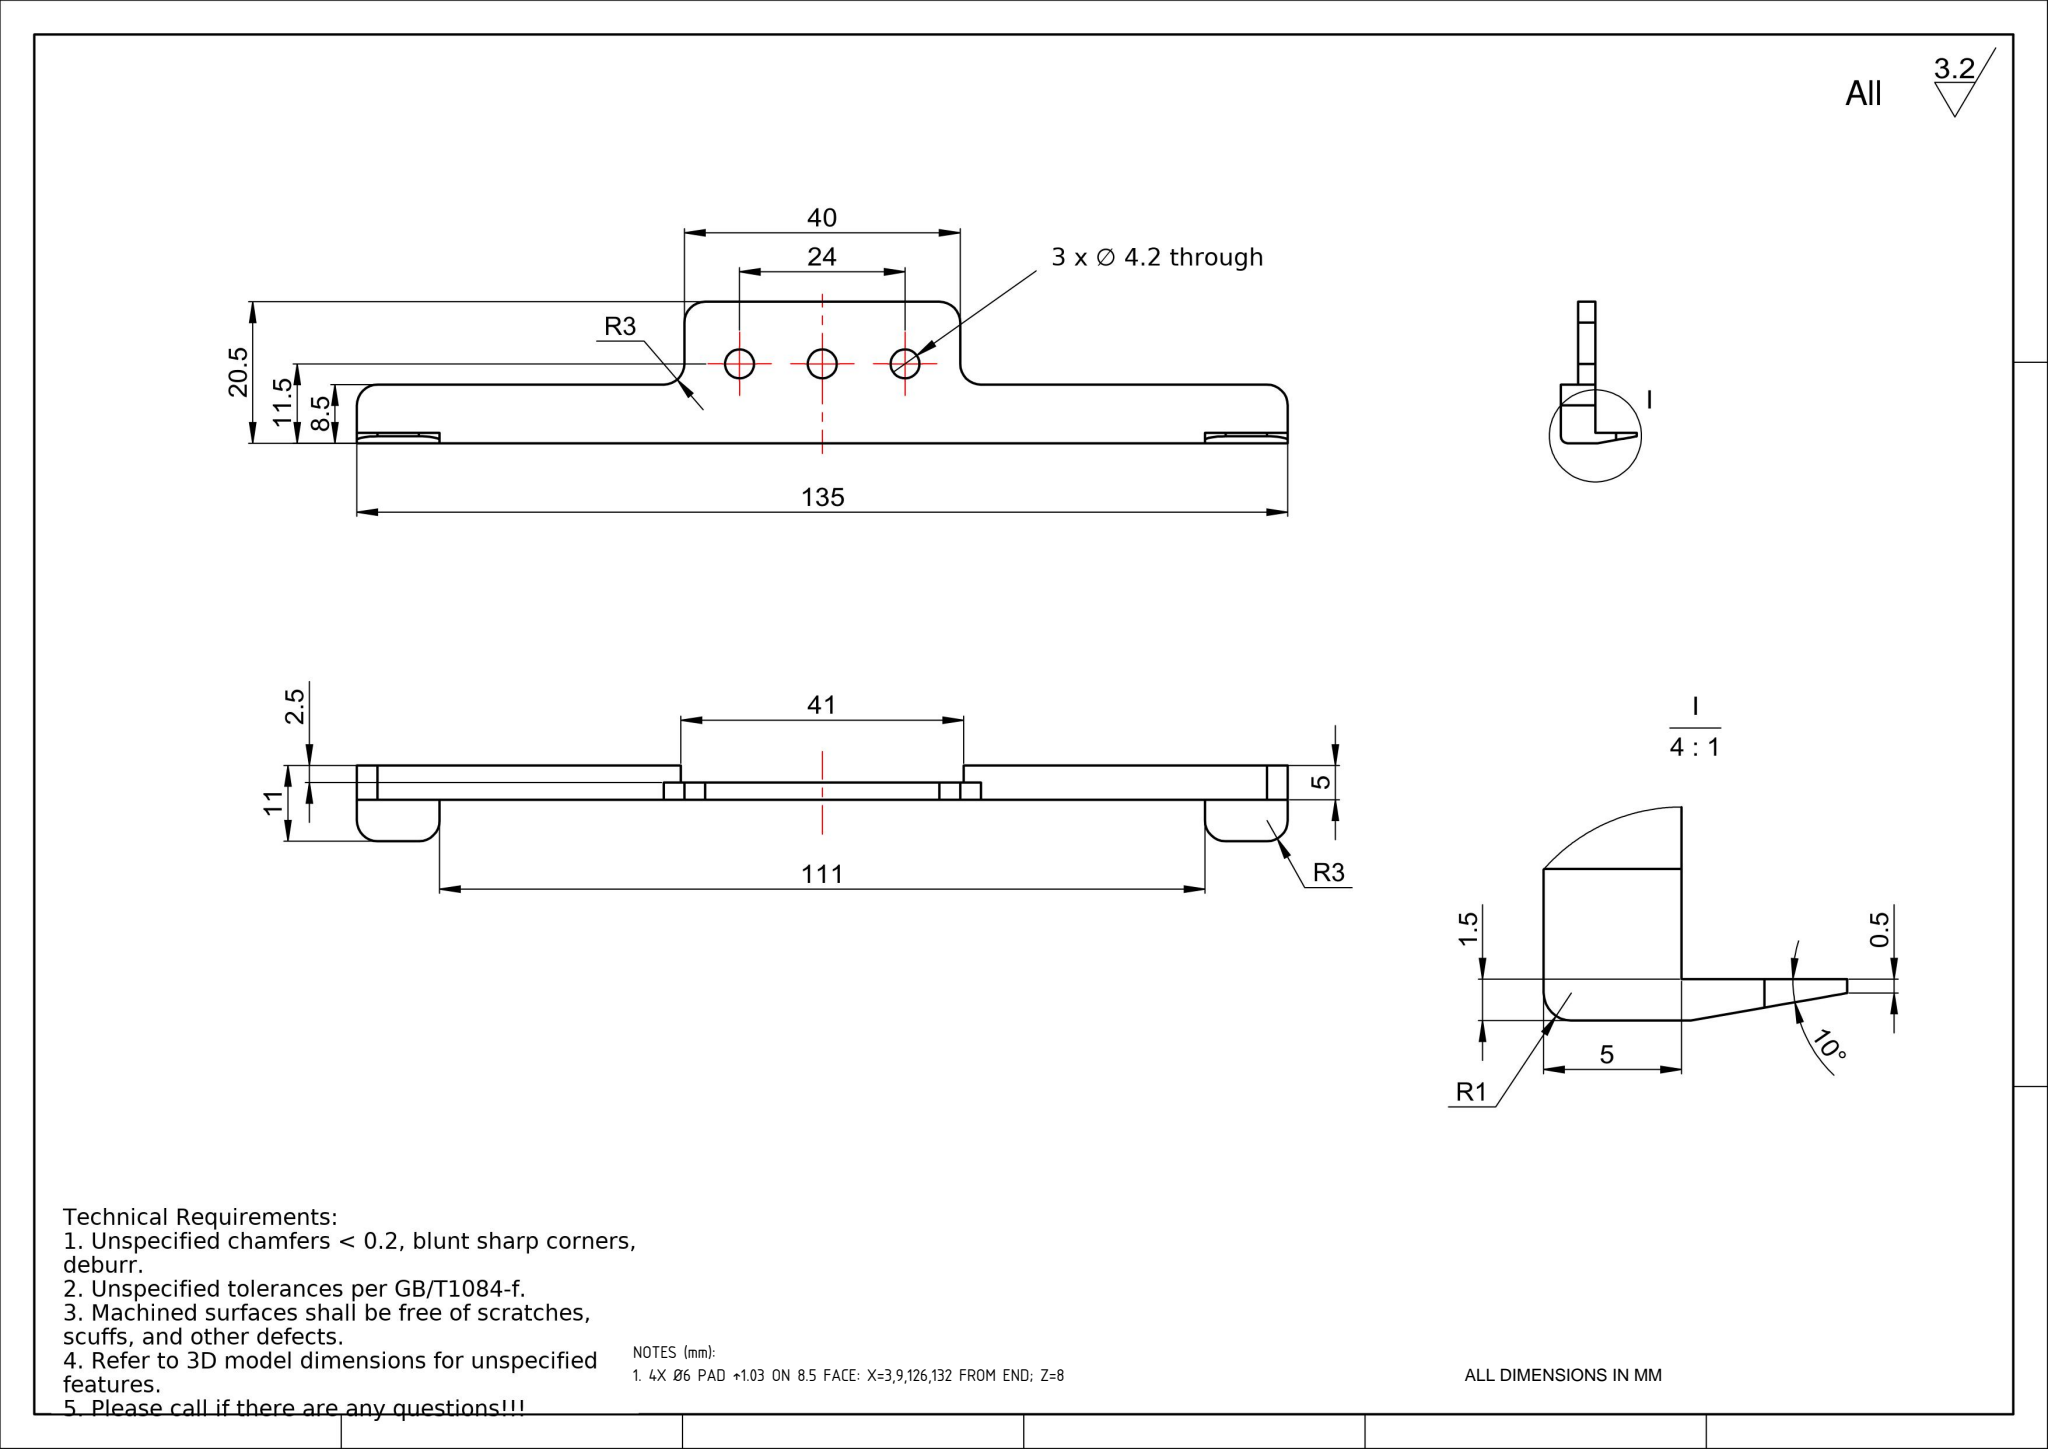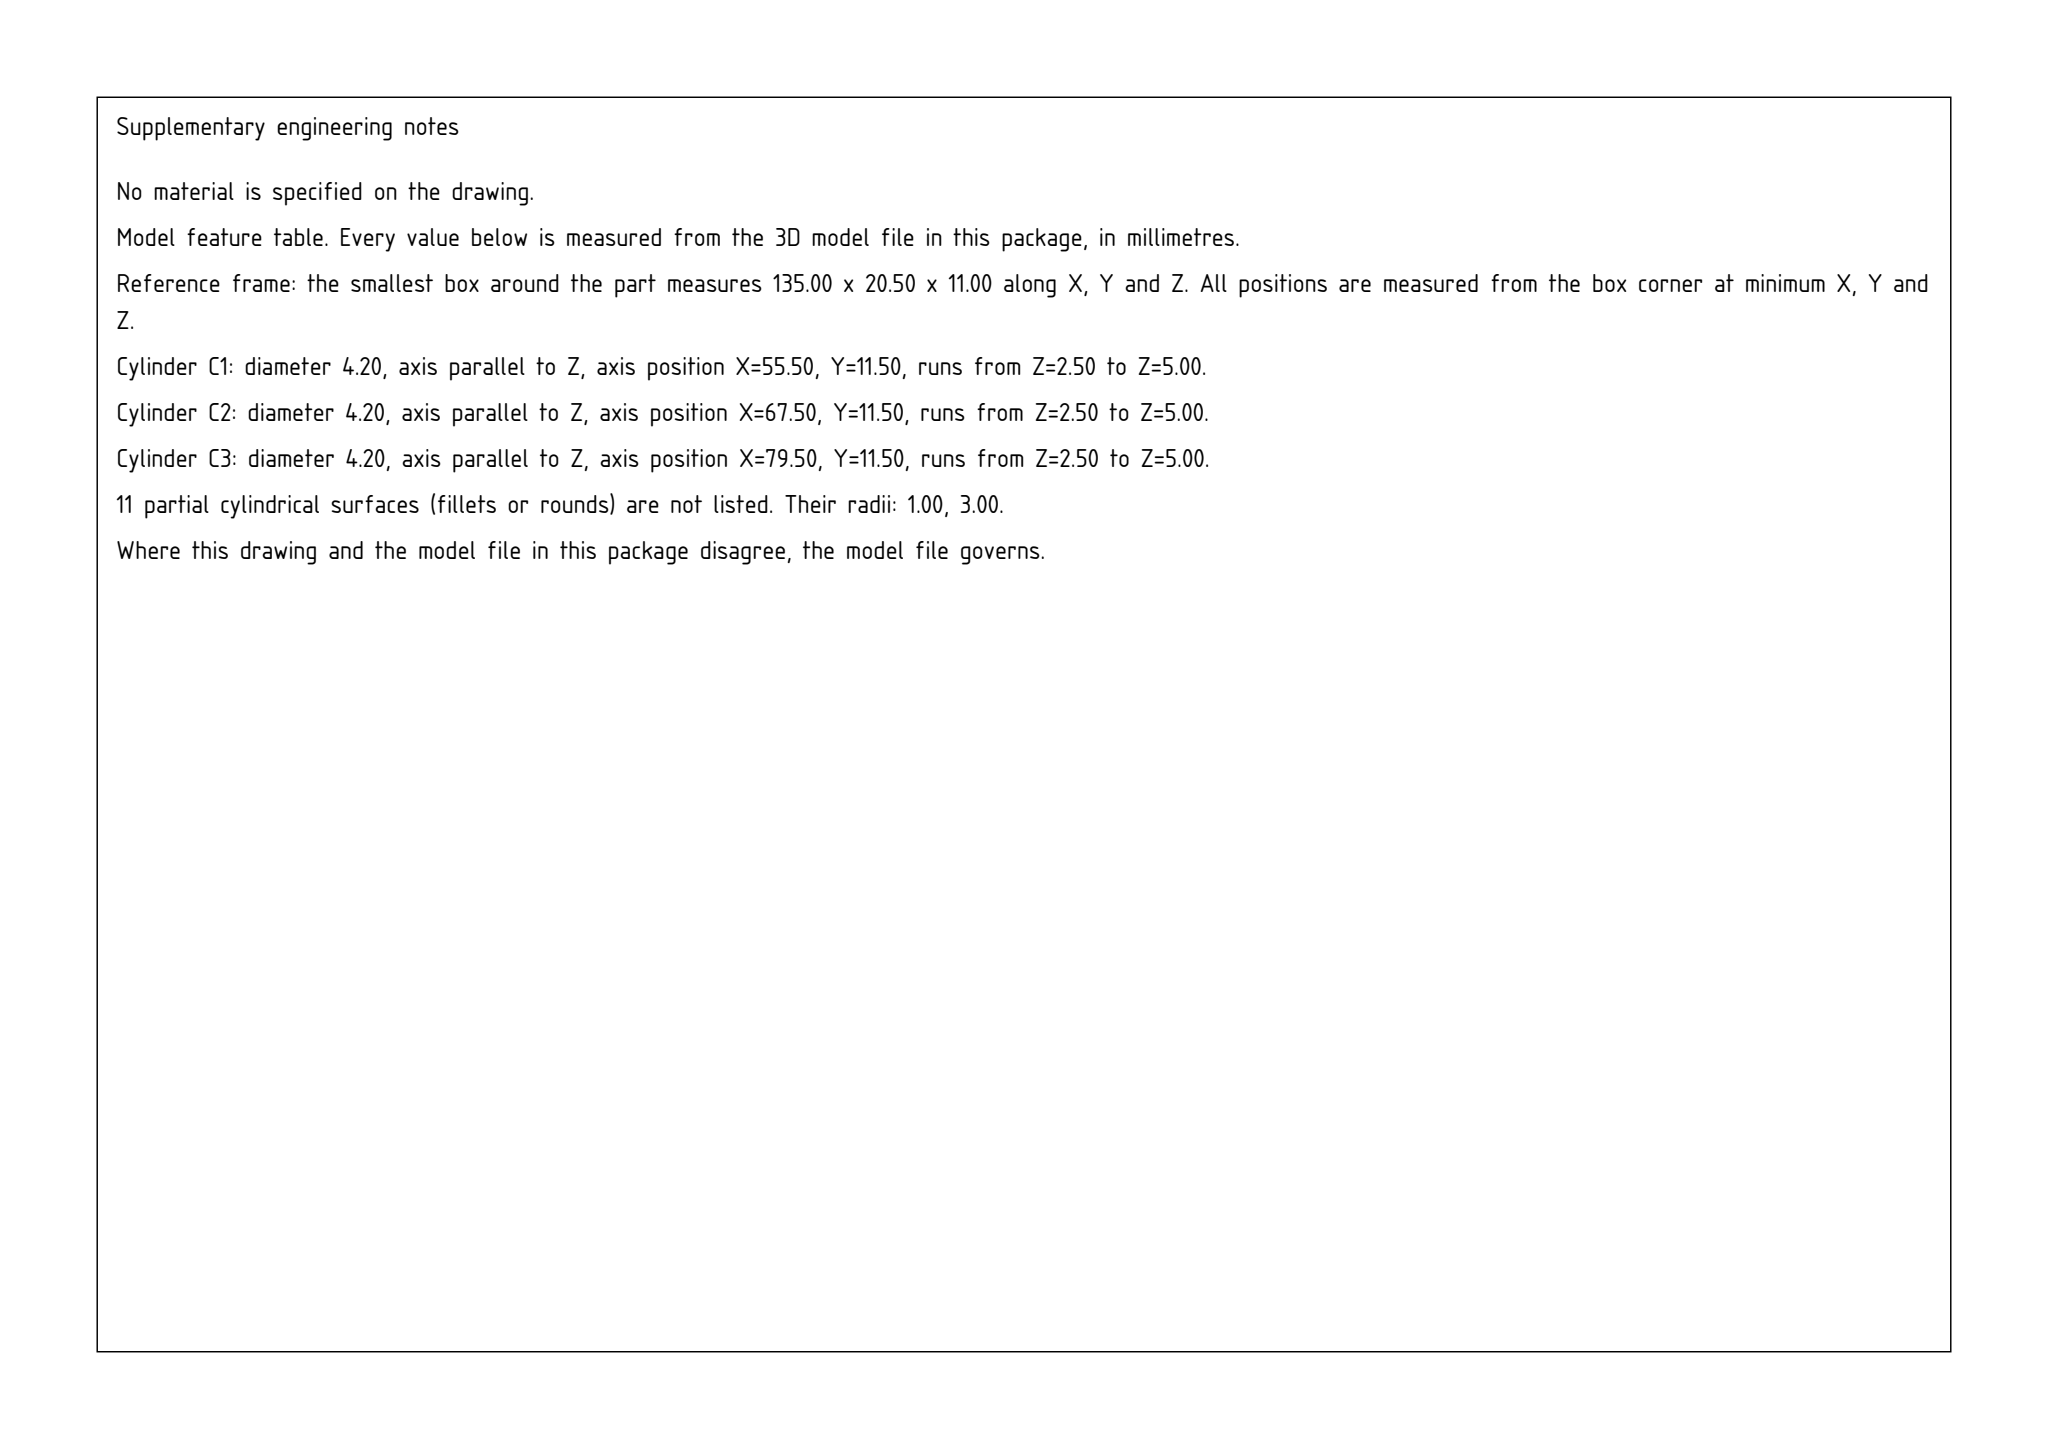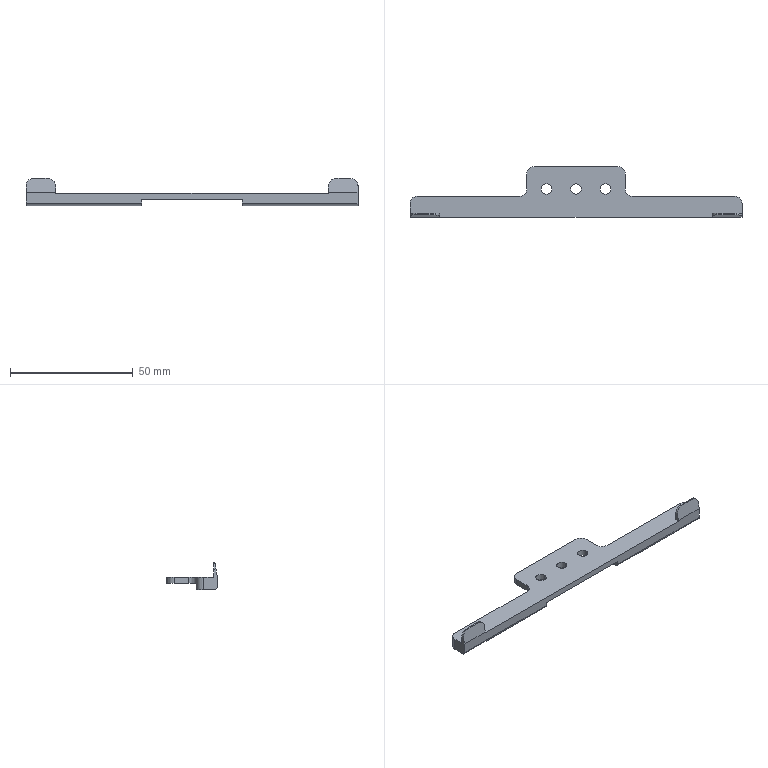Part | SolidWorks | mm | 1 solid | 40 faces | box 135 x 20.5 x 11 mm | volume 6066 mm3 | plane 22 | cylinder 18 | commonest cylinder face diameters 6 x10 4.2 x6 2 x2
Drawing notes:
4X Ø6 PAD ↑1.03 ON 8.5 FACE: X=3,9,126,132 FROM END; Z=8 | from the solid: cylinders dia 6.0 axis y, len 1.03, at (x=3,9,126,132; z=8), base on y=8.5 flange face; bbox 135x20.5x11